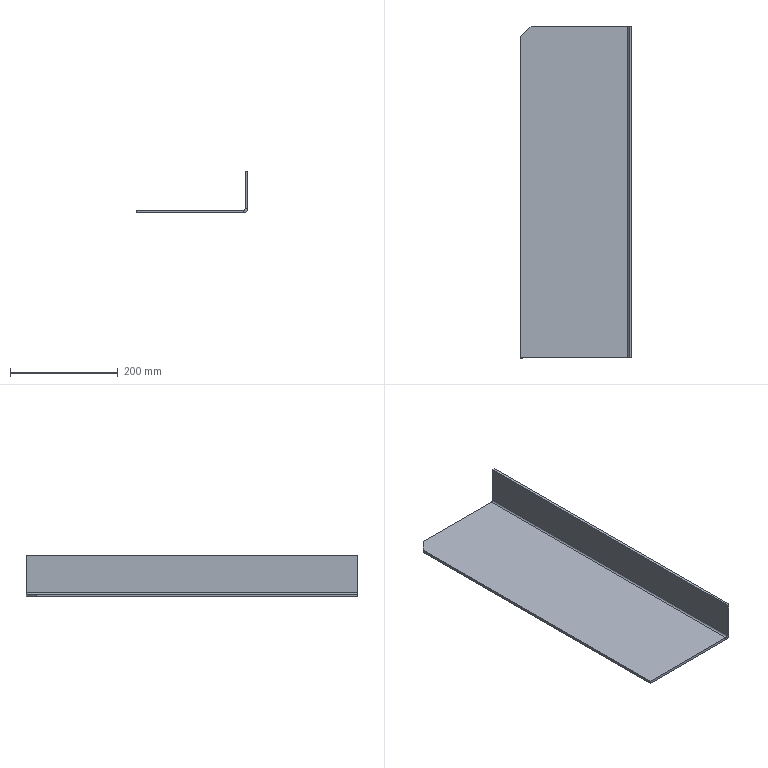Component | SolidWorks | FrontStiffener,Left-1 | 1 solid | 15 faces | box 206.64 x 615 x 77.36 mm | volume 849668 mm3 | plane 13 | cylinder 2 | commonest cylinder face diameters 6 x1 16 x1 | material Q235
STEP:
#1=CARTESIAN_POINT('',(-46.319,70.373,110.484));
#2=VERTEX_POINT('',#1);
#3=CARTESIAN_POINT('',(-46.319,70.373,107.753));
#4=VERTEX_POINT('',#3);
#5=CARTESIAN_POINT('',(-46.319,70.373,110.484));
#6=DIRECTION('',(0.,-0.,-1.));
#7=VECTOR('',#6,39.37);
#8=LINE('',#5,#7);
#9=EDGE_CURVE('',#2,#4,#8,.T.);
#10=ORIENTED_EDGE('',*,*,#9,.T.);
#11=CARTESIAN_POINT('',(-46.123,70.373,107.753));
#12=VERTEX_POINT('',#11);
#13=CARTESIAN_POINT('',(-46.319,70.373,107.753));
#14=DIRECTION('',(1.,0.,0.));
#15=VECTOR('',#14,39.37);
#16=LINE('',#13,#15);
#17=EDGE_CURVE('',#4,#12,#16,.T.);
#18=ORIENTED_EDGE('',*,*,#17,.T.);
#19=CARTESIAN_POINT('',(-46.123,70.373,110.484));
#20=VERTEX_POINT('',#19);
#21=CARTESIAN_POINT('',(-46.123,70.373,133.401));
#22=DIRECTION('',(0.,-0.,-1.));
#23=VECTOR('',#22,39.37);
#24=LINE('',#21,#23);
#25=EDGE_CURVE('',#20,#12,#24,.T.);
#26=ORIENTED_EDGE('',*,*,#25,.F.);
#27=CARTESIAN_POINT('',(-46.319,70.373,110.484));
#28=DIRECTION('',(-1.,-0.,-0.));
#29=VECTOR('',#28,39.37);
#30=LINE('',#27,#29);
#31=EDGE_CURVE('',#20,#2,#30,.T.);
#32=ORIENTED_EDGE('',*,*,#31,.T.);
#33=EDGE_LOOP('',(#10,#18,#26,#32));
#34=FACE_OUTER_BOUND('',#33,.T.);
#35=CARTESIAN_POINT('',(-46.319,70.373,110.484));
#36=DIRECTION('',(-0.,1.,-0.));
#37=DIRECTION('',(0.,-0.,-1.));
#38=AXIS2_PLACEMENT_3D('',#35,#36,#37);
#39=PLANE('',#38);
#40=ADVANCED_FACE('',(#34),#39,.F.);
#41=CARTESIAN_POINT('',(-46.123,94.586,110.484));
#42=VERTEX_POINT('',#41);
#43=CARTESIAN_POINT('',(-46.123,94.586,107.753));
#44=VERTEX_POINT('',#43);
#45=CARTESIAN_POINT('',(-46.123,94.586,133.401));
#46=DIRECTION('',(0.,-0.,-1.));
#47=VECTOR('',#46,39.37);
#48=LINE('',#45,#47);
#49=EDGE_CURVE('',#42,#44,#48,.T.);
#50=ORIENTED_EDGE('',*,*,#49,.T.);
#51=CARTESIAN_POINT('',(-46.319,94.586,107.753));
#52=VERTEX_POINT('',#51);
#53=CARTESIAN_POINT('',(-46.319,94.586,107.753));
#54=DIRECTION('',(-1.,-0.,-0.));
#55=VECTOR('',#54,39.37);
#56=LINE('',#53,#55);
#57=EDGE_CURVE('',#44,#52,#56,.T.);
#58=ORIENTED_EDGE('',*,*,#57,.T.);
#59=CARTESIAN_POINT('',(-46.319,94.586,110.484));
#60=VERTEX_POINT('',#59);
#61=CARTESIAN_POINT('',(-46.319,94.586,110.484));
#62=DIRECTION('',(0.,-0.,-1.));
#63=VECTOR('',#62,39.37);
#64=LINE('',#61,#63);
#65=EDGE_CURVE('',#60,#52,#64,.T.);
#66=ORIENTED_EDGE('',*,*,#65,.F.);
#67=CARTESIAN_POINT('',(-46.319,94.586,110.484));
#68=DIRECTION('',(-1.,-0.,-0.));
#69=VECTOR('',#68,39.37);
#70=LINE('',#67,#69);
#71=EDGE_CURVE('',#42,#60,#70,.T.);
#72=ORIENTED_EDGE('',*,*,#71,.F.);
#73=EDGE_LOOP('',(#50,#58,#66,#72));
#74=FACE_OUTER_BOUND('',#73,.T.);
#75=CARTESIAN_POINT('',(-46.319,94.586,110.484));
#76=DIRECTION('',(-0.,1.,-0.));
#77=DIRECTION('',(0.,-0.,-1.));
#78=AXIS2_PLACEMENT_3D('',#75,#76,#77);
#79=PLANE('',#78);
#80=ADVANCED_FACE('',(#74),#79,.T.);
#81=ORIENTED_EDGE('',*,*,#65,.T.);
#82=CARTESIAN_POINT('',(-46.319,101.625,107.753));
#83=DIRECTION('',(0.,-1.,0.));
#84=VECTOR('',#83,39.37);
#85=LINE('',#82,#84);
#86=EDGE_CURVE('',#52,#4,#85,.T.);
#87=ORIENTED_EDGE('',*,*,#86,.T.);
#88=ORIENTED_EDGE('',*,*,#9,.F.);
#89=CARTESIAN_POINT('',(-46.319,94.586,110.484));
#90=DIRECTION('',(0.,-1.,0.));
#91=VECTOR('',#90,39.37);
#92=LINE('',#89,#91);
#93=EDGE_CURVE('',#60,#2,#92,.T.);
#94=ORIENTED_EDGE('',*,*,#93,.F.);
#95=EDGE_LOOP('',(#81,#87,#88,#94));
#96=FACE_OUTER_BOUND('',#95,.T.);
#97=CARTESIAN_POINT('',(-46.319,101.625,133.401));
#98=DIRECTION('',(-1.,-0.,-0.));
#99=DIRECTION('',(-0.,1.,-0.));
#100=AXIS2_PLACEMENT_3D('',#97,#98,#99);
#101=PLANE('',#100);
#102=ADVANCED_FACE('',(#96),#101,.T.);
#103=ORIENTED_EDGE('',*,*,#31,.F.);
#104=CARTESIAN_POINT('',(-46.123,101.625,110.484));
#105=DIRECTION('',(0.,-1.,0.));
#106=VECTOR('',#105,39.37);
#107=LINE('',#104,#106);
#108=EDGE_CURVE('',#42,#20,#107,.T.);
#109=ORIENTED_EDGE('',*,*,#108,.F.);
#110=ORIENTED_EDGE('',*,*,#71,.T.);
#111=ORIENTED_EDGE('',*,*,#93,.T.);
#112=EDGE_LOOP('',(#103,#109,#110,#111));
#113=FACE_OUTER_BOUND('',#112,.T.);
#114=CARTESIAN_POINT('',(-46.319,94.586,110.484));
#115=DIRECTION('',(0.,-0.,-1.));
#116=DIRECTION('',(0.,-1.,0.));
#117=AXIS2_PLACEMENT_3D('',#114,#115,#116);
#118=PLANE('',#117);
#119=ADVANCED_FACE('',(#113),#118,.F.);
#120=CARTESIAN_POINT('',(-46.123,101.625,107.753));
#121=DIRECTION('',(0.,-1.,0.));
#122=VECTOR('',#121,39.37);
#123=LINE('',#120,#122);
#124=EDGE_CURVE('',#44,#12,#123,.T.);
#125=ORIENTED_EDGE('',*,*,#124,.F.);
#126=ORIENTED_EDGE('',*,*,#49,.F.);
#127=ORIENTED_EDGE('',*,*,#108,.T.);
#128=ORIENTED_EDGE('',*,*,#25,.T.);
#129=EDGE_LOOP('',(#125,#126,#127,#128));
#130=FACE_OUTER_BOUND('',#129,.T.);
#131=CARTESIAN_POINT('',(-46.123,101.625,133.401));
#132=DIRECTION('',(-1.,-0.,-0.));
#133=DIRECTION('',(-0.,1.,-0.));
#134=AXIS2_PLACEMENT_3D('',#131,#132,#133);
#135=PLANE('',#134);
#136=ADVANCED_FACE('',(#130),#135,.F.);
#137=CARTESIAN_POINT('',(-54.258,93.798,107.438));
#138=VERTEX_POINT('',#137);
#139=CARTESIAN_POINT('',(-54.258,70.373,107.438));
#140=VERTEX_POINT('',#139);
#141=CARTESIAN_POINT('',(-54.258,101.625,107.438));
#142=DIRECTION('',(0.,-1.,0.));
#143=VECTOR('',#142,39.37);
#144=LINE('',#141,#143);
#145=EDGE_CURVE('',#138,#140,#144,.T.);
#146=ORIENTED_EDGE('',*,*,#145,.T.);
#147=CARTESIAN_POINT('',(-54.258,70.373,107.635));
#148=VERTEX_POINT('',#147);
#149=CARTESIAN_POINT('',(-54.258,70.373,107.635));
#150=DIRECTION('',(-0.,0.,1.));
#151=VECTOR('',#150,39.37);
#152=LINE('',#149,#151);
#153=EDGE_CURVE('',#140,#148,#152,.T.);
#154=ORIENTED_EDGE('',*,*,#153,.T.);
#155=CARTESIAN_POINT('',(-54.258,93.798,107.635));
#156=VERTEX_POINT('',#155);
#157=CARTESIAN_POINT('',(-54.258,93.798,107.635));
#158=DIRECTION('',(0.,-1.,0.));
#159=VECTOR('',#158,39.37);
#160=LINE('',#157,#159);
#161=EDGE_CURVE('',#156,#148,#160,.T.);
#162=ORIENTED_EDGE('',*,*,#161,.F.);
#163=CARTESIAN_POINT('',(-54.258,93.798,107.635));
#164=DIRECTION('',(-0.,0.,1.));
#165=VECTOR('',#164,39.37);
#166=LINE('',#163,#165);
#167=EDGE_CURVE('',#138,#156,#166,.T.);
#168=ORIENTED_EDGE('',*,*,#167,.F.);
#169=EDGE_LOOP('',(#146,#154,#162,#168));
#170=FACE_OUTER_BOUND('',#169,.T.);
#171=CARTESIAN_POINT('',(-54.258,93.798,107.635));
#172=DIRECTION('',(-1.,-0.,-0.));
#173=DIRECTION('',(0.,-1.,0.));
#174=AXIS2_PLACEMENT_3D('',#171,#172,#173);
#175=PLANE('',#174);
#176=ADVANCED_FACE('',(#170),#175,.T.);
#177=CARTESIAN_POINT('',(-53.471,94.586,107.438));
#178=VERTEX_POINT('',#177);
#179=CARTESIAN_POINT('',(-53.471,94.586,107.635));
#180=VERTEX_POINT('',#179);
#181=CARTESIAN_POINT('',(-53.471,94.586,107.635));
#182=DIRECTION('',(-0.,0.,1.));
#183=VECTOR('',#182,39.37);
#184=LINE('',#181,#183);
#185=EDGE_CURVE('',#178,#180,#184,.T.);
#186=ORIENTED_EDGE('',*,*,#185,.F.);
#187=CARTESIAN_POINT('',(-53.471,94.586,107.438));
#188=DIRECTION('',(-0.7071,-0.7071,-0.));
#189=VECTOR('',#188,39.37);
#190=LINE('',#187,#189);
#191=EDGE_CURVE('',#178,#138,#190,.T.);
#192=ORIENTED_EDGE('',*,*,#191,.T.);
#193=ORIENTED_EDGE('',*,*,#167,.T.);
#194=CARTESIAN_POINT('',(-53.471,94.586,107.635));
#195=DIRECTION('',(-0.7071,-0.7071,-0.));
#196=VECTOR('',#195,39.37);
#197=LINE('',#194,#196);
#198=EDGE_CURVE('',#180,#156,#197,.T.);
#199=ORIENTED_EDGE('',*,*,#198,.F.);
#200=EDGE_LOOP('',(#186,#192,#193,#199));
#201=FACE_OUTER_BOUND('',#200,.T.);
#202=CARTESIAN_POINT('',(-53.471,94.586,107.635));
#203=DIRECTION('',(-0.7071,0.7071,-0.));
#204=DIRECTION('',(-0.7071,-0.7071,-0.));
#205=AXIS2_PLACEMENT_3D('',#202,#203,#204);
#206=PLANE('',#205);
#207=ADVANCED_FACE('',(#201),#206,.T.);
#208=CARTESIAN_POINT('',(-46.438,94.586,107.635));
#209=VERTEX_POINT('',#208);
#210=CARTESIAN_POINT('',(-46.438,70.373,107.635));
#211=VERTEX_POINT('',#210);
#212=CARTESIAN_POINT('',(-46.438,101.625,107.635));
#213=DIRECTION('',(0.,-1.,0.));
#214=VECTOR('',#213,39.37);
#215=LINE('',#212,#214);
#216=EDGE_CURVE('',#209,#211,#215,.T.);
#217=ORIENTED_EDGE('',*,*,#216,.F.);
#218=CARTESIAN_POINT('',(-43.367,94.586,107.635));
#219=DIRECTION('',(-1.,-0.,-0.));
#220=VECTOR('',#219,39.37);
#221=LINE('',#218,#220);
#222=EDGE_CURVE('',#209,#180,#221,.T.);
#223=ORIENTED_EDGE('',*,*,#222,.T.);
#224=ORIENTED_EDGE('',*,*,#198,.T.);
#225=ORIENTED_EDGE('',*,*,#161,.T.);
#226=CARTESIAN_POINT('',(-43.367,70.373,107.635));
#227=DIRECTION('',(-1.,-0.,-0.));
#228=VECTOR('',#227,39.37);
#229=LINE('',#226,#228);
#230=EDGE_CURVE('',#211,#148,#229,.T.);
#231=ORIENTED_EDGE('',*,*,#230,.F.);
#232=EDGE_LOOP('',(#217,#223,#224,#225,#231));
#233=FACE_OUTER_BOUND('',#232,.T.);
#234=CARTESIAN_POINT('',(-20.449,101.625,107.635));
#235=DIRECTION('',(-0.,0.,1.));
#236=DIRECTION('',(-0.,1.,-0.));
#237=AXIS2_PLACEMENT_3D('',#234,#235,#236);
#238=PLANE('',#237);
#239=ADVANCED_FACE('',(#233),#238,.T.);
#240=CARTESIAN_POINT('',(-46.438,94.586,107.438));
#241=VERTEX_POINT('',#240);
#242=CARTESIAN_POINT('',(-46.438,94.586,107.635));
#243=DIRECTION('',(-0.,0.,1.));
#244=VECTOR('',#243,39.37);
#245=LINE('',#242,#244);
#246=EDGE_CURVE('',#241,#209,#245,.T.);
#247=ORIENTED_EDGE('',*,*,#246,.F.);
#248=CARTESIAN_POINT('',(-20.449,94.586,107.438));
#249=DIRECTION('',(-1.,-0.,-0.));
#250=VECTOR('',#249,39.37);
#251=LINE('',#248,#250);
#252=EDGE_CURVE('',#241,#178,#251,.T.);
#253=ORIENTED_EDGE('',*,*,#252,.T.);
#254=ORIENTED_EDGE('',*,*,#185,.T.);
#255=ORIENTED_EDGE('',*,*,#222,.F.);
#256=EDGE_LOOP('',(#247,#253,#254,#255));
#257=FACE_OUTER_BOUND('',#256,.T.);
#258=CARTESIAN_POINT('',(-43.367,94.586,107.635));
#259=DIRECTION('',(-0.,1.,-0.));
#260=DIRECTION('',(-1.,-0.,-0.));
#261=AXIS2_PLACEMENT_3D('',#258,#259,#260);
#262=PLANE('',#261);
#263=ADVANCED_FACE('',(#257),#262,.T.);
#264=ORIENTED_EDGE('',*,*,#252,.F.);
#265=CARTESIAN_POINT('',(-46.438,70.373,107.438));
#266=VERTEX_POINT('',#265);
#267=CARTESIAN_POINT('',(-46.438,101.625,107.438));
#268=DIRECTION('',(0.,-1.,0.));
#269=VECTOR('',#268,39.37);
#270=LINE('',#267,#269);
#271=EDGE_CURVE('',#241,#266,#270,.T.);
#272=ORIENTED_EDGE('',*,*,#271,.T.);
#273=CARTESIAN_POINT('',(-20.449,70.373,107.438));
#274=DIRECTION('',(-1.,-0.,-0.));
#275=VECTOR('',#274,39.37);
#276=LINE('',#273,#275);
#277=EDGE_CURVE('',#266,#140,#276,.T.);
#278=ORIENTED_EDGE('',*,*,#277,.T.);
#279=ORIENTED_EDGE('',*,*,#145,.F.);
#280=ORIENTED_EDGE('',*,*,#191,.F.);
#281=EDGE_LOOP('',(#264,#272,#278,#279,#280));
#282=FACE_OUTER_BOUND('',#281,.T.);
#283=CARTESIAN_POINT('',(-20.449,101.625,107.438));
#284=DIRECTION('',(-0.,0.,1.));
#285=DIRECTION('',(-0.,1.,-0.));
#286=AXIS2_PLACEMENT_3D('',#283,#284,#285);
#287=PLANE('',#286);
#288=ADVANCED_FACE('',(#282),#287,.F.);
#289=CARTESIAN_POINT('',(-46.438,70.373,107.635));
#290=DIRECTION('',(0.,-0.,-1.));
#291=VECTOR('',#290,39.37);
#292=LINE('',#289,#291);
#293=EDGE_CURVE('',#211,#266,#292,.T.);
#294=ORIENTED_EDGE('',*,*,#293,.F.);
#295=ORIENTED_EDGE('',*,*,#230,.T.);
#296=ORIENTED_EDGE('',*,*,#153,.F.);
#297=ORIENTED_EDGE('',*,*,#277,.F.);
#298=EDGE_LOOP('',(#294,#295,#296,#297));
#299=FACE_OUTER_BOUND('',#298,.T.);
#300=CARTESIAN_POINT('',(-43.367,70.373,107.635));
#301=DIRECTION('',(-0.,1.,-0.));
#302=DIRECTION('',(-1.,-0.,-0.));
#303=AXIS2_PLACEMENT_3D('',#300,#301,#302);
#304=PLANE('',#303);
#305=ADVANCED_FACE('',(#299),#304,.F.);
#306=ORIENTED_EDGE('',*,*,#57,.F.);
#307=CARTESIAN_POINT('',(-46.438,94.586,107.753));
#308=DIRECTION('',(-0.,1.,-0.));
#309=DIRECTION('',(0.,0.,-1.));
#310=AXIS2_PLACEMENT_3D('',#307,#308,#309);
#311=CIRCLE('',#310,0.315);
#312=EDGE_CURVE('',#44,#241,#311,.T.);
#313=ORIENTED_EDGE('',*,*,#312,.T.);
#314=ORIENTED_EDGE('',*,*,#246,.T.);
#315=CARTESIAN_POINT('',(-46.438,94.586,107.753));
#316=DIRECTION('',(-0.,1.,-0.));
#317=DIRECTION('',(0.,0.,-1.));
#318=AXIS2_PLACEMENT_3D('',#315,#316,#317);
#319=CIRCLE('',#318,0.1181);
#320=EDGE_CURVE('',#52,#209,#319,.T.);
#321=ORIENTED_EDGE('',*,*,#320,.F.);
#322=EDGE_LOOP('',(#306,#313,#314,#321));
#323=FACE_OUTER_BOUND('',#322,.T.);
#324=CARTESIAN_POINT('',(-46.438,94.586,107.753));
#325=DIRECTION('',(0.,-1.,0.));
#326=DIRECTION('',(-0.,0.,1.));
#327=AXIS2_PLACEMENT_3D('',#324,#325,#326);
#328=PLANE('',#327);
#329=ADVANCED_FACE('',(#323),#328,.F.);
#330=CARTESIAN_POINT('',(-46.438,70.373,107.753));
#331=DIRECTION('',(0.,-1.,0.));
#332=DIRECTION('',(0.,0.,-1.));
#333=AXIS2_PLACEMENT_3D('',#330,#331,#332);
#334=CIRCLE('',#333,0.315);
#335=EDGE_CURVE('',#266,#12,#334,.T.);
#336=ORIENTED_EDGE('',*,*,#335,.T.);
#337=ORIENTED_EDGE('',*,*,#17,.F.);
#338=CARTESIAN_POINT('',(-46.438,70.373,107.753));
#339=DIRECTION('',(0.,-1.,0.));
#340=DIRECTION('',(0.,0.,-1.));
#341=AXIS2_PLACEMENT_3D('',#338,#339,#340);
#342=CIRCLE('',#341,0.1181);
#343=EDGE_CURVE('',#211,#4,#342,.T.);
#344=ORIENTED_EDGE('',*,*,#343,.F.);
#345=ORIENTED_EDGE('',*,*,#293,.T.);
#346=EDGE_LOOP('',(#336,#337,#344,#345));
#347=FACE_OUTER_BOUND('',#346,.T.);
#348=CARTESIAN_POINT('',(-46.438,70.373,107.753));
#349=DIRECTION('',(-0.,1.,-0.));
#350=DIRECTION('',(0.,-0.,-1.));
#351=AXIS2_PLACEMENT_3D('',#348,#349,#350);
#352=PLANE('',#351);
#353=ADVANCED_FACE('',(#347),#352,.F.);
#354=ORIENTED_EDGE('',*,*,#216,.T.);
#355=ORIENTED_EDGE('',*,*,#343,.T.);
#356=ORIENTED_EDGE('',*,*,#86,.F.);
#357=ORIENTED_EDGE('',*,*,#320,.T.);
#358=EDGE_LOOP('',(#354,#355,#356,#357));
#359=FACE_OUTER_BOUND('',#358,.T.);
#360=CARTESIAN_POINT('',(-46.438,58.264,107.753));
#361=DIRECTION('',(-0.,1.,-0.));
#362=DIRECTION('',(0.,0.,-1.));
#363=AXIS2_PLACEMENT_3D('',#360,#361,#362);
#364=CYLINDRICAL_SURFACE('',#363,0.1181);
#365=ADVANCED_FACE('',(#359),#364,.F.);
#366=ORIENTED_EDGE('',*,*,#271,.F.);
#367=ORIENTED_EDGE('',*,*,#312,.F.);
#368=ORIENTED_EDGE('',*,*,#124,.T.);
#369=ORIENTED_EDGE('',*,*,#335,.F.);
#370=EDGE_LOOP('',(#366,#367,#368,#369));
#371=FACE_OUTER_BOUND('',#370,.T.);
#372=CARTESIAN_POINT('',(-46.438,58.264,107.753));
#373=DIRECTION('',(-0.,1.,-0.));
#374=DIRECTION('',(0.,0.,-1.));
#375=AXIS2_PLACEMENT_3D('',#372,#373,#374);
#376=CYLINDRICAL_SURFACE('',#375,0.315);
#377=ADVANCED_FACE('',(#371),#376,.T.);
#378=CLOSED_SHELL('',(#40,#80,#102,#119,#136,#176,#207,#239,#263,#288,#305,#329,#353,#365,#377));
#379=MANIFOLD_SOLID_BREP('',#378);
#380=CARTESIAN_POINT('',(0.,0.,0.));
#381=DIRECTION('',(0.,0.,1.));
#382=DIRECTION('',(1.,0.,0.));
#383=AXIS2_PLACEMENT_3D('',#380,#381,#382);
#384=(LENGTH_UNIT()NAMED_UNIT(*)SI_UNIT($,.METRE.));
#385=LENGTH_MEASURE_WITH_UNIT(LENGTH_MEASURE(0.0254),#384);
#386=DIMENSIONAL_EXPONENTS(1.,0.,0.,0.,0.,0.,0.);
#387=(CONVERSION_BASED_UNIT('',#385)LENGTH_UNIT()NAMED_UNIT(#386));
#388=UNCERTAINTY_MEASURE_WITH_UNIT(LENGTH_MEASURE(0.00001),#387,'','');
#389=(NAMED_UNIT(*)PLANE_ANGLE_UNIT()SI_UNIT($,.RADIAN.));
#390=(NAMED_UNIT(*)SI_UNIT($,.STERADIAN.)SOLID_ANGLE_UNIT());
#391=(GEOMETRIC_REPRESENTATION_CONTEXT(3)GLOBAL_UNCERTAINTY_ASSIGNED_CONTEXT((#388))GLOBAL_UNIT_ASSIGNED_CONTEXT((#387,#389,#390))REPRESENTATION_CONTEXT('',''));
#392=ADVANCED_BREP_SHAPE_REPRESENTATION('',(#379,#383),#391);
#393=COLOUR_RGB('',0.7922,0.8196,0.9333);
#394=FILL_AREA_STYLE_COLOUR('',#393);
#395=FILL_AREA_STYLE('',(#394));
#396=SURFACE_STYLE_FILL_AREA(#395);
#397=SURFACE_SIDE_STYLE('',(#396));
#398=SURFACE_STYLE_USAGE(.BOTH.,#397);
#399=PRESENTATION_STYLE_ASSIGNMENT((#398));
#400=STYLED_ITEM('',(#399),#379);
#401=(LENGTH_UNIT()NAMED_UNIT(*)SI_UNIT($,.METRE.));
#402=LENGTH_MEASURE_WITH_UNIT(LENGTH_MEASURE(0.0254),#401);
#403=DIMENSIONAL_EXPONENTS(1.,0.,0.,0.,0.,0.,0.);
#404=(CONVERSION_BASED_UNIT('',#402)LENGTH_UNIT()NAMED_UNIT(#403));
#405=UNCERTAINTY_MEASURE_WITH_UNIT(LENGTH_MEASURE(0.00001),#404,'','');
#406=(NAMED_UNIT(*)PLANE_ANGLE_UNIT()SI_UNIT($,.RADIAN.));
#407=(NAMED_UNIT(*)SI_UNIT($,.STERADIAN.)SOLID_ANGLE_UNIT());
#408=(GEOMETRIC_REPRESENTATION_CONTEXT(3)GLOBAL_UNCERTAINTY_ASSIGNED_CONTEXT((#405))GLOBAL_UNIT_ASSIGNED_CONTEXT((#404,#406,#407))REPRESENTATION_CONTEXT('',''));
#409=MECHANICAL_DESIGN_GEOMETRIC_PRESENTATION_REPRESENTATION('',(#400),#408);
#410=PRESENTATION_LAYER_ASSIGNMENT('','',(#400));